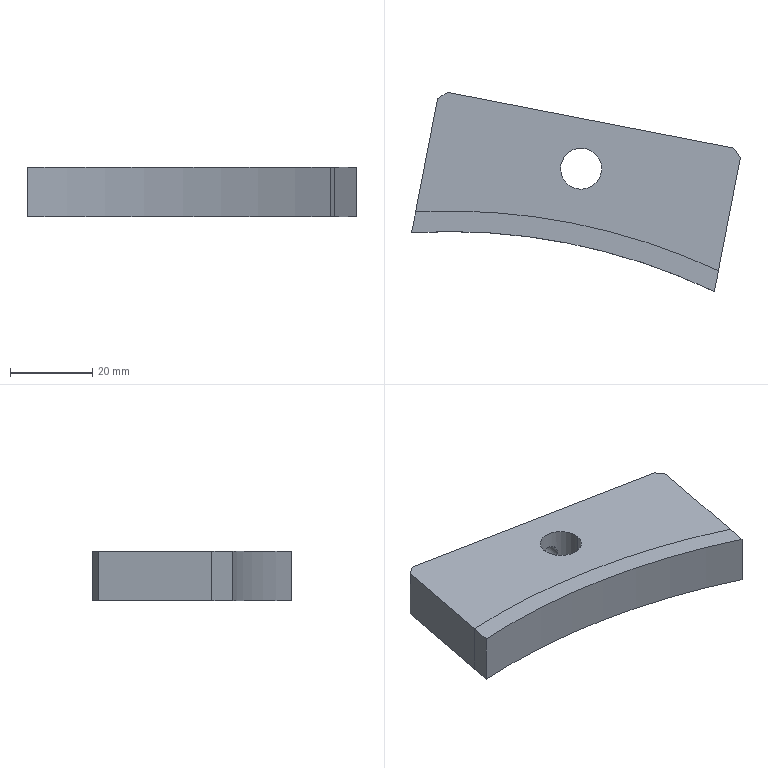Component | SolidWorks | JYTBJ-HeaderPlateBrakePad-1 | 2 solids | 18 faces | box 79.95 x 48.45 x 12 mm | volume 27686 mm3 | plane 11 | cylinder 7 | commonest cylinder face diameters 310 x2 4.2 x2 10 x2 300 x1
build123d program:
from build123d import *

# Parameters (mm, degrees)
BOSS_EXTRUDE1_DEPTH = 12
SKETCH2_R           = 5
CUT_EXTRUDE1_DEPTH  = 12
BOSS_EXTRUDE2_DEPTH = 12
CHAMFER1_SIZE       = 2


with BuildPart() as part:
    # Sketch1 → Boss-Extrude1 (new body)
    with BuildSketch(Plane.XY):
        with BuildLine():
            Line((-13.101, 22.851), (61.899, 22.851))
            Line((61.899, 22.851), (61.899, -7.149))
            ThreePointArc((61.899, -7.149), (24.399, -2.544), (-13.101, -7.149))
            Line((-13.101, -7.149), (-13.101, 22.851))
        make_face()
    extrude(amount=BOSS_EXTRUDE1_DEPTH)

    # Sketch2 → Cut-Extrude1 (cut)
    with BuildSketch(Plane.XY.offset(12)):
        with Locations((24.399, 10.851)):
            Circle(SKETCH2_R)
    extrude(amount=-CUT_EXTRUDE1_DEPTH, mode=Mode.SUBTRACT)

    # Sketch4 → M5 Tapped Hole1 (revolve, cut)
    with BuildSketch(Plane(origin=(24.399, 22.851, 6), x_dir=(0, 0, 1), z_dir=(1, 0, 0))):
        Polygon((0, 0), (0, 15.262), (2.1, 14), (2.1, 0), align=None)
    revolve(axis=Axis((24.399, 29.201, 6), (0, -1, 0)), mode=Mode.SUBTRACT)

    # Chamfer1
    chamfer1_edges = [part.edges().sort_by_distance(p)[0] for p in [
        (-13.101, 22.851, 6),
        (61.899, 22.851, 6),
    ]]
    chamfer(chamfer1_edges, length=CHAMFER1_SIZE)


with BuildPart() as body_2:
    # Sketch3 → Boss-Extrude2 (new body)
    with BuildSketch(Plane.XY.offset(12)):
        with BuildLine():
            Line((-13.101, -7.149), (-13.101, -12.307))
            ThreePointArc((-13.101, -12.307), (24.399, -7.544), (61.899, -12.307))
            Line((61.899, -12.307), (61.899, -7.149))
            ThreePointArc((61.899, -7.149), (24.399, -2.544), (-13.101, -7.149))
        make_face()
    extrude(amount=-BOSS_EXTRUDE2_DEPTH)


solid = Compound([part.part, body_2.part])

# Placed as in the assembly
solid = solid.moved(Location((9.701, 259.155, 38.5), (0, 0, -11.011)))
STEP:
#1=COLOUR_RGB('',0.7922,0.8196,0.9333);
#2=FILL_AREA_STYLE_COLOUR('',#1);
#3=FILL_AREA_STYLE('',(#2));
#4=SURFACE_STYLE_FILL_AREA(#3);
#5=SURFACE_SIDE_STYLE('',(#4));
#6=SURFACE_STYLE_USAGE(.BOTH.,#5);
#7=PRESENTATION_STYLE_ASSIGNMENT((#6));
#8=CARTESIAN_POINT('',(2.72,9.461,1.988));
#9=VERTEX_POINT('',#8);
#10=CARTESIAN_POINT('',(-0.1781,10.025,1.988));
#11=VERTEX_POINT('',#10);
#12=CARTESIAN_POINT('',(0.1402,3.931,1.988));
#13=DIRECTION('',(-0.,-0.,1.));
#14=DIRECTION('',(0.9816,-0.191,0.));
#15=AXIS2_PLACEMENT_3D('',#12,#13,#14);
#16=CIRCLE('',#15,6.102);
#17=EDGE_CURVE('',#9,#11,#16,.T.);
#18=ORIENTED_EDGE('',*,*,#17,.F.);
#19=CARTESIAN_POINT('',(2.72,9.461,1.516));
#20=VERTEX_POINT('',#19);
#21=CARTESIAN_POINT('',(2.72,9.461,1.516));
#22=DIRECTION('',(-0.,-0.,1.));
#23=VECTOR('',#22,39.37);
#24=LINE('',#21,#23);
#25=EDGE_CURVE('',#20,#9,#24,.T.);
#26=ORIENTED_EDGE('',*,*,#25,.F.);
#27=CARTESIAN_POINT('',(-0.1781,10.025,1.516));
#28=VERTEX_POINT('',#27);
#29=CARTESIAN_POINT('',(0.1402,3.931,1.516));
#30=DIRECTION('',(-0.,-0.,1.));
#31=DIRECTION('',(0.9816,-0.191,0.));
#32=AXIS2_PLACEMENT_3D('',#29,#30,#31);
#33=CIRCLE('',#32,6.102);
#34=EDGE_CURVE('',#20,#28,#33,.T.);
#35=ORIENTED_EDGE('',*,*,#34,.T.);
#36=CARTESIAN_POINT('',(-0.1781,10.025,1.516));
#37=DIRECTION('',(-0.,-0.,1.));
#38=VECTOR('',#37,39.37);
#39=LINE('',#36,#38);
#40=EDGE_CURVE('',#28,#11,#39,.T.);
#41=ORIENTED_EDGE('',*,*,#40,.T.);
#42=EDGE_LOOP('',(#18,#26,#35,#41));
#43=FACE_OUTER_BOUND('',#42,.T.);
#44=CARTESIAN_POINT('',(0.1402,3.931,1.516));
#45=DIRECTION('',(-0.,-0.,1.));
#46=DIRECTION('',(0.9816,-0.191,0.));
#47=AXIS2_PLACEMENT_3D('',#44,#45,#46);
#48=CYLINDRICAL_SURFACE('',#47,6.102);
#49=ADVANCED_FACE('',(#43),#48,.T.);
#50=CARTESIAN_POINT('',(2.682,9.262,1.988));
#51=VERTEX_POINT('',#50);
#52=CARTESIAN_POINT('',(2.72,9.461,1.988));
#53=DIRECTION('',(0.191,0.9816,0.));
#54=VECTOR('',#53,39.37);
#55=LINE('',#52,#54);
#56=EDGE_CURVE('',#51,#9,#55,.T.);
#57=ORIENTED_EDGE('',*,*,#56,.F.);
#58=CARTESIAN_POINT('',(2.682,9.262,1.516));
#59=VERTEX_POINT('',#58);
#60=CARTESIAN_POINT('',(2.682,9.262,1.516));
#61=DIRECTION('',(-0.,-0.,1.));
#62=VECTOR('',#61,39.37);
#63=LINE('',#60,#62);
#64=EDGE_CURVE('',#59,#51,#63,.T.);
#65=ORIENTED_EDGE('',*,*,#64,.F.);
#66=CARTESIAN_POINT('',(2.72,9.461,1.516));
#67=DIRECTION('',(0.191,0.9816,0.));
#68=VECTOR('',#67,39.37);
#69=LINE('',#66,#68);
#70=EDGE_CURVE('',#59,#20,#69,.T.);
#71=ORIENTED_EDGE('',*,*,#70,.T.);
#72=ORIENTED_EDGE('',*,*,#25,.T.);
#73=EDGE_LOOP('',(#57,#65,#71,#72));
#74=FACE_OUTER_BOUND('',#73,.T.);
#75=CARTESIAN_POINT('',(2.72,9.461,1.516));
#76=DIRECTION('',(0.9816,-0.191,0.));
#77=DIRECTION('',(0.,0.,-1.));
#78=AXIS2_PLACEMENT_3D('',#75,#76,#77);
#79=PLANE('',#78);
#80=ADVANCED_FACE('',(#74),#79,.T.);
#81=CARTESIAN_POINT('',(-0.2169,9.826,1.988));
#82=VERTEX_POINT('',#81);
#83=CARTESIAN_POINT('',(0.1402,3.931,1.988));
#84=DIRECTION('',(0.,0.,-1.));
#85=DIRECTION('',(0.9816,-0.191,0.));
#86=AXIS2_PLACEMENT_3D('',#83,#84,#85);
#87=CIRCLE('',#86,5.906);
#88=EDGE_CURVE('',#82,#51,#87,.T.);
#89=ORIENTED_EDGE('',*,*,#88,.F.);
#90=CARTESIAN_POINT('',(-0.2169,9.826,1.516));
#91=VERTEX_POINT('',#90);
#92=CARTESIAN_POINT('',(-0.2169,9.826,1.516));
#93=DIRECTION('',(-0.,-0.,1.));
#94=VECTOR('',#93,39.37);
#95=LINE('',#92,#94);
#96=EDGE_CURVE('',#91,#82,#95,.T.);
#97=ORIENTED_EDGE('',*,*,#96,.F.);
#98=CARTESIAN_POINT('',(0.1402,3.931,1.516));
#99=DIRECTION('',(0.,0.,-1.));
#100=DIRECTION('',(0.9816,-0.191,0.));
#101=AXIS2_PLACEMENT_3D('',#98,#99,#100);
#102=CIRCLE('',#101,5.906);
#103=EDGE_CURVE('',#91,#59,#102,.T.);
#104=ORIENTED_EDGE('',*,*,#103,.T.);
#105=ORIENTED_EDGE('',*,*,#64,.T.);
#106=EDGE_LOOP('',(#89,#97,#104,#105));
#107=FACE_OUTER_BOUND('',#106,.T.);
#108=CARTESIAN_POINT('',(0.1402,3.931,1.516));
#109=DIRECTION('',(-0.,-0.,1.));
#110=DIRECTION('',(0.9816,-0.191,0.));
#111=AXIS2_PLACEMENT_3D('',#108,#109,#110);
#112=CYLINDRICAL_SURFACE('',#111,5.906);
#113=ADVANCED_FACE('',(#107),#112,.F.);
#114=CARTESIAN_POINT('',(-0.1781,10.025,1.988));
#115=DIRECTION('',(-0.191,-0.9816,-0.));
#116=VECTOR('',#115,39.37);
#117=LINE('',#114,#116);
#118=EDGE_CURVE('',#11,#82,#117,.T.);
#119=ORIENTED_EDGE('',*,*,#118,.F.);
#120=ORIENTED_EDGE('',*,*,#40,.F.);
#121=CARTESIAN_POINT('',(-0.1781,10.025,1.516));
#122=DIRECTION('',(-0.191,-0.9816,-0.));
#123=VECTOR('',#122,39.37);
#124=LINE('',#121,#123);
#125=EDGE_CURVE('',#28,#91,#124,.T.);
#126=ORIENTED_EDGE('',*,*,#125,.T.);
#127=ORIENTED_EDGE('',*,*,#96,.T.);
#128=EDGE_LOOP('',(#119,#120,#126,#127));
#129=FACE_OUTER_BOUND('',#128,.T.);
#130=CARTESIAN_POINT('',(-0.1781,10.025,1.516));
#131=DIRECTION('',(-0.9816,0.191,-0.));
#132=DIRECTION('',(-0.191,-0.9816,-0.));
#133=AXIS2_PLACEMENT_3D('',#130,#131,#132);
#134=PLANE('',#133);
#135=ADVANCED_FACE('',(#129),#134,.T.);
#136=ORIENTED_EDGE('',*,*,#34,.F.);
#137=ORIENTED_EDGE('',*,*,#70,.F.);
#138=ORIENTED_EDGE('',*,*,#103,.F.);
#139=ORIENTED_EDGE('',*,*,#125,.F.);
#140=EDGE_LOOP('',(#136,#137,#138,#139));
#141=FACE_OUTER_BOUND('',#140,.T.);
#142=CARTESIAN_POINT('',(0.1402,3.931,1.516));
#143=DIRECTION('',(-0.,-0.,1.));
#144=DIRECTION('',(0.9816,-0.191,0.));
#145=AXIS2_PLACEMENT_3D('',#142,#143,#144);
#146=PLANE('',#145);
#147=ADVANCED_FACE('',(#141),#146,.F.);
#148=ORIENTED_EDGE('',*,*,#17,.T.);
#149=ORIENTED_EDGE('',*,*,#118,.T.);
#150=ORIENTED_EDGE('',*,*,#88,.T.);
#151=ORIENTED_EDGE('',*,*,#56,.T.);
#152=EDGE_LOOP('',(#148,#149,#150,#151));
#153=FACE_OUTER_BOUND('',#152,.T.);
#154=CARTESIAN_POINT('',(0.1402,3.931,1.988));
#155=DIRECTION('',(-0.,-0.,1.));
#156=DIRECTION('',(0.9816,-0.191,0.));
#157=AXIS2_PLACEMENT_3D('',#154,#155,#156);
#158=PLANE('',#157);
#159=ADVANCED_FACE('',(#153),#158,.T.);
#160=CLOSED_SHELL('',(#49,#80,#113,#135,#147,#159));
#161=MANIFOLD_SOLID_BREP('',#160);
#162=STYLED_ITEM('',(#7),#161);
#163=PRESENTATION_LAYER_ASSIGNMENT('','',(#162));
#164=COLOUR_RGB('',0.7922,0.8196,0.9333);
#165=FILL_AREA_STYLE_COLOUR('',#164);
#166=FILL_AREA_STYLE('',(#165));
#167=SURFACE_STYLE_FILL_AREA(#166);
#168=SURFACE_SIDE_STYLE('',(#167));
#169=SURFACE_STYLE_USAGE(.BOTH.,#168);
#170=PRESENTATION_STYLE_ASSIGNMENT((#169));
#171=CARTESIAN_POINT('',(1.444,10.632,1.669));
#172=VERTEX_POINT('',#171);
#173=CARTESIAN_POINT('',(1.444,10.632,1.835));
#174=VERTEX_POINT('',#173);
#175=CARTESIAN_POINT('',(1.444,10.632,1.669));
#176=CARTESIAN_POINT('',(1.439,10.633,1.669));
#177=CARTESIAN_POINT('',(1.433,10.634,1.67));
#178=CARTESIAN_POINT('',(1.423,10.635,1.672));
#179=CARTESIAN_POINT('',(1.417,10.635,1.674));
#180=CARTESIAN_POINT('',(1.407,10.636,1.678));
#181=CARTESIAN_POINT('',(1.402,10.636,1.68));
#182=CARTESIAN_POINT('',(1.393,10.635,1.686));
#183=CARTESIAN_POINT('',(1.389,10.635,1.69));
#184=CARTESIAN_POINT('',(1.381,10.634,1.697));
#185=CARTESIAN_POINT('',(1.377,10.634,1.701));
#186=CARTESIAN_POINT('',(1.371,10.633,1.71));
#187=CARTESIAN_POINT('',(1.368,10.632,1.715));
#188=CARTESIAN_POINT('',(1.364,10.631,1.725));
#189=CARTESIAN_POINT('',(1.362,10.631,1.73));
#190=CARTESIAN_POINT('',(1.36,10.63,1.741));
#191=CARTESIAN_POINT('',(1.359,10.63,1.746));
#192=CARTESIAN_POINT('',(1.359,10.63,1.763));
#193=CARTESIAN_POINT('',(1.362,10.631,1.774));
#194=CARTESIAN_POINT('',(1.368,10.632,1.789));
#195=CARTESIAN_POINT('',(1.371,10.633,1.794));
#196=CARTESIAN_POINT('',(1.377,10.634,1.802));
#197=CARTESIAN_POINT('',(1.381,10.634,1.807));
#198=CARTESIAN_POINT('',(1.389,10.635,1.814));
#199=CARTESIAN_POINT('',(1.393,10.635,1.818));
#200=CARTESIAN_POINT('',(1.402,10.636,1.824));
#201=CARTESIAN_POINT('',(1.407,10.636,1.826));
#202=CARTESIAN_POINT('',(1.417,10.635,1.83));
#203=CARTESIAN_POINT('',(1.423,10.635,1.832));
#204=CARTESIAN_POINT('',(1.433,10.634,1.834));
#205=CARTESIAN_POINT('',(1.439,10.633,1.835));
#206=CARTESIAN_POINT('',(1.444,10.632,1.835));
#207=B_SPLINE_CURVE_WITH_KNOTS('',3,(#175,#176,#177,#178,#179,#180,#181,#182,#183,#184,#185,#186,#187,#188,#189,#190,#191,#192,#193,#194,#195,#196,#197,#198,#199,#200,#201,#202,#203,#204,#205,#206),.UNSPECIFIED.,.F.,.F.,(4,2,2,2,2,2,2,2,2,2,2,2,2,2,2,4),(0.006644,0.007058,0.007473,0.007888,0.008303,0.008718,0.009133,0.009548,0.009963,0.01079,0.01121,0.01162,0.01204,0.01245,0.01287,0.01328),.UNSPECIFIED.);
#208=EDGE_CURVE('',#172,#174,#207,.T.);
#209=ORIENTED_EDGE('',*,*,#208,.F.);
#210=CARTESIAN_POINT('',(1.497,10.903,1.669));
#211=VERTEX_POINT('',#210);
#212=CARTESIAN_POINT('',(1.497,10.903,1.669));
#213=DIRECTION('',(0.191,0.9816,0.));
#214=VECTOR('',#213,39.37);
#215=LINE('',#212,#214);
#216=EDGE_CURVE('',#172,#211,#215,.T.);
#217=ORIENTED_EDGE('',*,*,#216,.T.);
#218=CARTESIAN_POINT('',(1.497,10.903,1.835));
#219=VERTEX_POINT('',#218);
#220=CARTESIAN_POINT('',(1.497,10.903,1.752));
#221=DIRECTION('',(0.191,0.9816,0.));
#222=DIRECTION('',(0.,0.,1.));
#223=AXIS2_PLACEMENT_3D('',#220,#221,#222);
#224=CIRCLE('',#223,0.08268);
#225=EDGE_CURVE('',#211,#219,#224,.T.);
#226=ORIENTED_EDGE('',*,*,#225,.T.);
#227=CARTESIAN_POINT('',(1.497,10.903,1.835));
#228=DIRECTION('',(0.191,0.9816,0.));
#229=VECTOR('',#228,39.37);
#230=LINE('',#227,#229);
#231=EDGE_CURVE('',#174,#219,#230,.T.);
#232=ORIENTED_EDGE('',*,*,#231,.F.);
#233=EDGE_LOOP('',(#209,#217,#226,#232));
#234=FACE_OUTER_BOUND('',#233,.T.);
#235=CARTESIAN_POINT('',(1.497,10.903,1.752));
#236=DIRECTION('',(0.191,0.9816,0.));
#237=DIRECTION('',(0.,0.,1.));
#238=AXIS2_PLACEMENT_3D('',#235,#236,#237);
#239=CYLINDRICAL_SURFACE('',#238,0.08268);
#240=ADVANCED_FACE('',(#234),#239,.F.);
#241=CARTESIAN_POINT('',(1.213,10.476,1.516));
#242=VERTEX_POINT('',#241);
#243=CARTESIAN_POINT('',(1.6,10.401,1.516));
#244=VERTEX_POINT('',#243);
#245=CARTESIAN_POINT('',(1.406,10.439,1.516));
#246=DIRECTION('',(-0.,-0.,1.));
#247=DIRECTION('',(0.9816,-0.191,0.));
#248=AXIS2_PLACEMENT_3D('',#245,#246,#247);
#249=CIRCLE('',#248,0.1969);
#250=EDGE_CURVE('',#242,#244,#249,.T.);
#251=ORIENTED_EDGE('',*,*,#250,.F.);
#252=CARTESIAN_POINT('',(1.213,10.476,1.988));
#253=VERTEX_POINT('',#252);
#254=CARTESIAN_POINT('',(1.213,10.476,1.516));
#255=DIRECTION('',(-0.,-0.,1.));
#256=VECTOR('',#255,39.37);
#257=LINE('',#254,#256);
#258=EDGE_CURVE('',#242,#253,#257,.T.);
#259=ORIENTED_EDGE('',*,*,#258,.T.);
#260=CARTESIAN_POINT('',(1.6,10.401,1.988));
#261=VERTEX_POINT('',#260);
#262=CARTESIAN_POINT('',(1.406,10.439,1.988));
#263=DIRECTION('',(-0.,-0.,1.));
#264=DIRECTION('',(0.9816,-0.191,0.));
#265=AXIS2_PLACEMENT_3D('',#262,#263,#264);
#266=CIRCLE('',#265,0.1969);
#267=EDGE_CURVE('',#253,#261,#266,.T.);
#268=ORIENTED_EDGE('',*,*,#267,.T.);
#269=CARTESIAN_POINT('',(1.6,10.401,1.516));
#270=DIRECTION('',(-0.,-0.,1.));
#271=VECTOR('',#270,39.37);
#272=LINE('',#269,#271);
#273=EDGE_CURVE('',#244,#261,#272,.T.);
#274=ORIENTED_EDGE('',*,*,#273,.F.);
#275=EDGE_LOOP('',(#251,#259,#268,#274));
#276=FACE_OUTER_BOUND('',#275,.T.);
#277=CARTESIAN_POINT('',(1.406,10.439,1.516));
#278=DIRECTION('',(-0.,-0.,1.));
#279=DIRECTION('',(0.9816,-0.191,0.));
#280=AXIS2_PLACEMENT_3D('',#277,#278,#279);
#281=CYLINDRICAL_SURFACE('',#280,0.1969);
#282=ADVANCED_FACE('',(#276),#281,.F.);
#283=CARTESIAN_POINT('',(0.03244,11.107,1.988));
#284=VERTEX_POINT('',#283);
#285=CARTESIAN_POINT('',(-0.1781,10.025,1.988));
#286=VERTEX_POINT('',#285);
#287=CARTESIAN_POINT('',(0.04748,11.185,1.988));
#288=DIRECTION('',(-0.191,-0.9816,-0.));
#289=VECTOR('',#288,39.37);
#290=LINE('',#287,#289);
#291=EDGE_CURVE('',#284,#286,#290,.T.);
#292=ORIENTED_EDGE('',*,*,#291,.F.);
#293=CARTESIAN_POINT('',(0.03244,11.107,1.516));
#294=VERTEX_POINT('',#293);
#295=CARTESIAN_POINT('',(0.03244,11.107,1.988));
#296=DIRECTION('',(0.,0.,-1.));
#297=VECTOR('',#296,39.37);
#298=LINE('',#295,#297);
#299=EDGE_CURVE('',#284,#294,#298,.T.);
#300=ORIENTED_EDGE('',*,*,#299,.T.);
#301=CARTESIAN_POINT('',(-0.1781,10.025,1.516));
#302=VERTEX_POINT('',#301);
#303=CARTESIAN_POINT('',(0.04748,11.185,1.516));
#304=DIRECTION('',(-0.191,-0.9816,-0.));
#305=VECTOR('',#304,39.37);
#306=LINE('',#303,#305);
#307=EDGE_CURVE('',#294,#302,#306,.T.);
#308=ORIENTED_EDGE('',*,*,#307,.T.);
#309=CARTESIAN_POINT('',(-0.1781,10.025,1.988));
#310=DIRECTION('',(0.,0.,-1.));
#311=VECTOR('',#310,39.37);
#312=LINE('',#309,#311);
#313=EDGE_CURVE('',#286,#302,#312,.T.);
#314=ORIENTED_EDGE('',*,*,#313,.F.);
#315=EDGE_LOOP('',(#292,#300,#308,#314));
#316=FACE_OUTER_BOUND('',#315,.T.);
#317=CARTESIAN_POINT('',(0.04748,11.185,1.988));
#318=DIRECTION('',(0.9816,-0.191,0.));
#319=DIRECTION('',(0.191,0.9816,0.));
#320=AXIS2_PLACEMENT_3D('',#317,#318,#319);
#321=PLANE('',#320);
#322=ADVANCED_FACE('',(#316),#321,.F.);
#323=CARTESIAN_POINT('',(2.72,9.461,1.516));
#324=VERTEX_POINT('',#323);
#325=CARTESIAN_POINT('',(0.1402,3.931,1.516));
#326=DIRECTION('',(0.,0.,-1.));
#327=DIRECTION('',(0.9816,-0.191,0.));
#328=AXIS2_PLACEMENT_3D('',#325,#326,#327);
#329=CIRCLE('',#328,6.102);
#330=EDGE_CURVE('',#302,#324,#329,.T.);
#331=ORIENTED_EDGE('',*,*,#330,.T.);
#332=CARTESIAN_POINT('',(2.72,9.461,1.988));
#333=VERTEX_POINT('',#332);
#334=CARTESIAN_POINT('',(2.72,9.461,1.988));
#335=DIRECTION('',(0.,0.,-1.));
#336=VECTOR('',#335,39.37);
#337=LINE('',#334,#336);
#338=EDGE_CURVE('',#333,#324,#337,.T.);
#339=ORIENTED_EDGE('',*,*,#338,.F.);
#340=CARTESIAN_POINT('',(0.1402,3.931,1.988));
#341=DIRECTION('',(0.,0.,-1.));
#342=DIRECTION('',(0.9816,-0.191,0.));
#343=AXIS2_PLACEMENT_3D('',#340,#341,#342);
#344=CIRCLE('',#343,6.102);
#345=EDGE_CURVE('',#286,#333,#344,.T.);
#346=ORIENTED_EDGE('',*,*,#345,.F.);
#347=ORIENTED_EDGE('',*,*,#313,.T.);
#348=EDGE_LOOP('',(#331,#339,#346,#347));
#349=FACE_OUTER_BOUND('',#348,.T.);
#350=CARTESIAN_POINT('',(0.1402,3.931,1.988));
#351=DIRECTION('',(0.,0.,-1.));
#352=DIRECTION('',(-0.9816,0.191,0.));
#353=AXIS2_PLACEMENT_3D('',#350,#351,#352);
#354=CYLINDRICAL_SURFACE('',#353,6.102);
#355=ADVANCED_FACE('',(#349),#354,.F.);
#356=CARTESIAN_POINT('',(2.931,10.543,1.516));
#357=VERTEX_POINT('',#356);
#358=CARTESIAN_POINT('',(2.946,10.621,1.516));
#359=DIRECTION('',(0.191,0.9816,0.));
#360=VECTOR('',#359,39.37);
#361=LINE('',#358,#360);
#362=EDGE_CURVE('',#324,#357,#361,.T.);
#363=ORIENTED_EDGE('',*,*,#362,.T.);
#364=CARTESIAN_POINT('',(2.931,10.543,1.988));
#365=VERTEX_POINT('',#364);
#366=CARTESIAN_POINT('',(2.931,10.543,1.988));
#367=DIRECTION('',(-0.,-0.,1.));
#368=VECTOR('',#367,39.37);
#369=LINE('',#366,#368);
#370=EDGE_CURVE('',#357,#365,#369,.T.);
#371=ORIENTED_EDGE('',*,*,#370,.T.);
#372=CARTESIAN_POINT('',(2.946,10.621,1.988));
#373=DIRECTION('',(0.191,0.9816,0.));
#374=VECTOR('',#373,39.37);
#375=LINE('',#372,#374);
#376=EDGE_CURVE('',#333,#365,#375,.T.);
#377=ORIENTED_EDGE('',*,*,#376,.F.);
#378=ORIENTED_EDGE('',*,*,#338,.T.);
#379=EDGE_LOOP('',(#363,#371,#377,#378));
#380=FACE_OUTER_BOUND('',#379,.T.);
#381=CARTESIAN_POINT('',(2.946,10.621,1.988));
#382=DIRECTION('',(-0.9816,0.191,-0.));
#383=DIRECTION('',(-0.,-0.,1.));
#384=AXIS2_PLACEMENT_3D('',#381,#382,#383);
#385=PLANE('',#384);
#386=ADVANCED_FACE('',(#380),#385,.F.);
#387=CARTESIAN_POINT('',(1.497,10.903,1.752));
#388=DIRECTION('',(0.191,0.9816,0.));
#389=DIRECTION('',(0.,0.,1.));
#390=AXIS2_PLACEMENT_3D('',#387,#388,#389);
#391=CIRCLE('',#390,0.08268);
#392=EDGE_CURVE('',#219,#211,#391,.T.);
#393=ORIENTED_EDGE('',*,*,#392,.F.);
#394=ORIENTED_EDGE('',*,*,#225,.F.);
#395=EDGE_LOOP('',(#393,#394));
#396=FACE_BOUND('',#395,.T.);
#397=CARTESIAN_POINT('',(2.869,10.636,1.988));
#398=VERTEX_POINT('',#397);
#399=CARTESIAN_POINT('',(0.1248,11.17,1.988));
#400=VERTEX_POINT('',#399);
#401=CARTESIAN_POINT('',(0.04748,11.185,1.988));
#402=DIRECTION('',(-0.9816,0.191,-0.));
#403=VECTOR('',#402,39.37);
#404=LINE('',#401,#403);
#405=EDGE_CURVE('',#398,#400,#404,.T.);
#406=ORIENTED_EDGE('',*,*,#405,.F.);
#407=CARTESIAN_POINT('',(2.869,10.636,1.516));
#408=VERTEX_POINT('',#407);
#409=CARTESIAN_POINT('',(2.869,10.636,1.988));
#410=DIRECTION('',(0.,0.,-1.));
#411=VECTOR('',#410,39.37);
#412=LINE('',#409,#411);
#413=EDGE_CURVE('',#398,#408,#412,.T.);
#414=ORIENTED_EDGE('',*,*,#413,.T.);
#415=CARTESIAN_POINT('',(0.1248,11.17,1.516));
#416=VERTEX_POINT('',#415);
#417=CARTESIAN_POINT('',(0.04748,11.185,1.516));
#418=DIRECTION('',(-0.9816,0.191,-0.));
#419=VECTOR('',#418,39.37);
#420=LINE('',#417,#419);
#421=EDGE_CURVE('',#408,#416,#420,.T.);
#422=ORIENTED_EDGE('',*,*,#421,.T.);
#423=CARTESIAN_POINT('',(0.1248,11.17,1.988));
#424=DIRECTION('',(-0.,-0.,1.));
#425=VECTOR('',#424,39.37);
#426=LINE('',#423,#425);
#427=EDGE_CURVE('',#416,#400,#426,.T.);
#428=ORIENTED_EDGE('',*,*,#427,.T.);
#429=EDGE_LOOP('',(#406,#414,#422,#428));
#430=FACE_OUTER_BOUND('',#429,.T.);
#431=CARTESIAN_POINT('',(0.04748,11.185,1.988));
#432=DIRECTION('',(-0.191,-0.9816,-0.));
#433=DIRECTION('',(0.,0.,-1.));
#434=AXIS2_PLACEMENT_3D('',#431,#432,#433);
#435=PLANE('',#434);
#436=ADVANCED_FACE('',(#396,#430),#435,.F.);
#437=CARTESIAN_POINT('',(1.406,10.439,1.988));
#438=DIRECTION('',(-0.,-0.,1.));
#439=DIRECTION('',(0.9816,-0.191,0.));
#440=AXIS2_PLACEMENT_3D('',#437,#438,#439);
#441=CIRCLE('',#440,0.1969);
#442=EDGE_CURVE('',#261,#253,#441,.T.);
#443=ORIENTED_EDGE('',*,*,#442,.F.);
#444=ORIENTED_EDGE('',*,*,#267,.F.);
#445=EDGE_LOOP('',(#443,#444));
#446=FACE_BOUND('',#445,.T.);
#447=ORIENTED_EDGE('',*,*,#376,.T.);
#448=CARTESIAN_POINT('',(5.124,7.291,1.988));
#449=DIRECTION('',(-0.559,0.8291,0.));
#450=VECTOR('',#449,39.37);
#451=LINE('',#448,#450);
#452=EDGE_CURVE('',#365,#398,#451,.T.);
#453=ORIENTED_EDGE('',*,*,#452,.T.);
#454=ORIENTED_EDGE('',*,*,#405,.T.);
#455=CARTESIAN_POINT('',(-3.22,8.915,1.988));
#456=DIRECTION('',(-0.8291,-0.559,-0.));
#457=VECTOR('',#456,39.37);
#458=LINE('',#455,#457);
#459=EDGE_CURVE('',#400,#284,#458,.T.);
#460=ORIENTED_EDGE('',*,*,#459,.T.);
#461=ORIENTED_EDGE('',*,*,#291,.T.);
#462=ORIENTED_EDGE('',*,*,#345,.T.);
#463=EDGE_LOOP('',(#447,#453,#454,#460,#461,#462));
#464=FACE_OUTER_BOUND('',#463,.T.);
#465=CARTESIAN_POINT('',(0.1402,3.931,1.988));
#466=DIRECTION('',(-0.,-0.,1.));
#467=DIRECTION('',(0.9816,-0.191,0.));
#468=AXIS2_PLACEMENT_3D('',#465,#466,#467);
#469=PLANE('',#468);
#470=ADVANCED_FACE('',(#446,#464),#469,.T.);
#471=CARTESIAN_POINT('',(1.406,10.439,1.516));
#472=DIRECTION('',(-0.,-0.,1.));
#473=DIRECTION('',(0.9816,-0.191,0.));
#474=AXIS2_PLACEMENT_3D('',#471,#472,#473);
#475=CIRCLE('',#474,0.1969);
#476=EDGE_CURVE('',#244,#242,#475,.T.);
#477=ORIENTED_EDGE('',*,*,#476,.T.);
#478=ORIENTED_EDGE('',*,*,#250,.T.);
#479=EDGE_LOOP('',(#477,#478));
#480=FACE_BOUND('',#479,.T.);
#481=ORIENTED_EDGE('',*,*,#421,.F.);
#482=CARTESIAN_POINT('',(2.869,10.636,1.516));
#483=DIRECTION('',(0.559,-0.8291,-0.));
#484=VECTOR('',#483,39.37);
#485=LINE('',#482,#484);
#486=EDGE_CURVE('',#408,#357,#485,.T.);
#487=ORIENTED_EDGE('',*,*,#486,.T.);
#488=ORIENTED_EDGE('',*,*,#362,.F.);
#489=ORIENTED_EDGE('',*,*,#330,.F.);
#490=ORIENTED_EDGE('',*,*,#307,.F.);
#491=CARTESIAN_POINT('',(0.03244,11.107,1.516));
#492=DIRECTION('',(0.8291,0.559,0.));
#493=VECTOR('',#492,39.37);
#494=LINE('',#491,#493);
#495=EDGE_CURVE('',#294,#416,#494,.T.);
#496=ORIENTED_EDGE('',*,*,#495,.T.);
#497=EDGE_LOOP('',(#481,#487,#488,#489,#490,#496));
#498=FACE_OUTER_BOUND('',#497,.T.);
#499=CARTESIAN_POINT('',(0.1402,3.931,1.516));
#500=DIRECTION('',(-0.,-0.,1.));
#501=DIRECTION('',(0.9816,-0.191,0.));
#502=AXIS2_PLACEMENT_3D('',#499,#500,#501);
#503=PLANE('',#502);
#504=ADVANCED_FACE('',(#480,#498),#503,.F.);
#505=ORIENTED_EDGE('',*,*,#258,.F.);
#506=ORIENTED_EDGE('',*,*,#476,.F.);
#507=ORIENTED_EDGE('',*,*,#273,.T.);
#508=ORIENTED_EDGE('',*,*,#442,.T.);
#509=EDGE_LOOP('',(#505,#506,#507,#508));
#510=FACE_OUTER_BOUND('',#509,.T.);
#511=CARTESIAN_POINT('',(1.444,10.632,1.835));
#512=CARTESIAN_POINT('',(1.449,10.631,1.835));
#513=CARTESIAN_POINT('',(1.455,10.63,1.834));
#514=CARTESIAN_POINT('',(1.465,10.627,1.832));
#515=CARTESIAN_POINT('',(1.47,10.625,1.83));
#516=CARTESIAN_POINT('',(1.48,10.622,1.826));
#517=CARTESIAN_POINT('',(1.484,10.62,1.824));
#518=CARTESIAN_POINT('',(1.492,10.616,1.818));
#519=CARTESIAN_POINT('',(1.496,10.614,1.814));
#520=CARTESIAN_POINT('',(1.507,10.608,1.803));
#521=CARTESIAN_POINT('',(1.512,10.605,1.794));
#522=CARTESIAN_POINT('',(1.518,10.601,1.779));
#523=CARTESIAN_POINT('',(1.519,10.6,1.774));
#524=CARTESIAN_POINT('',(1.521,10.599,1.763));
#525=CARTESIAN_POINT('',(1.522,10.598,1.757));
#526=CARTESIAN_POINT('',(1.522,10.598,1.747));
#527=CARTESIAN_POINT('',(1.521,10.599,1.741));
#528=CARTESIAN_POINT('',(1.519,10.6,1.73));
#529=CARTESIAN_POINT('',(1.518,10.601,1.725));
#530=CARTESIAN_POINT('',(1.514,10.604,1.715));
#531=CARTESIAN_POINT('',(1.512,10.605,1.71));
#532=CARTESIAN_POINT('',(1.506,10.608,1.701));
#533=CARTESIAN_POINT('',(1.503,10.61,1.697));
#534=CARTESIAN_POINT('',(1.496,10.614,1.69));
#535=CARTESIAN_POINT('',(1.492,10.616,1.686));
#536=CARTESIAN_POINT('',(1.484,10.62,1.68));
#537=CARTESIAN_POINT('',(1.48,10.622,1.678));
#538=CARTESIAN_POINT('',(1.465,10.627,1.672));
#539=CARTESIAN_POINT('',(1.455,10.63,1.669));
#540=CARTESIAN_POINT('',(1.444,10.632,1.669));
#541=B_SPLINE_CURVE_WITH_KNOTS('',3,(#511,#512,#513,#514,#515,#516,#517,#518,#519,#520,#521,#522,#523,#524,#525,#526,#527,#528,#529,#530,#531,#532,#533,#534,#535,#536,#537,#538,#539,#540),.UNSPECIFIED.,.F.,.F.,(4,2,2,2,2,2,2,2,2,2,2,2,2,2,4),(0.,0.0004152,0.0008304,0.001246,0.001661,0.002491,0.002907,0.003322,0.003737,0.004152,0.004567,0.004983,0.005398,0.005813,0.006644),.UNSPECIFIED.);
#542=EDGE_CURVE('',#174,#172,#541,.T.);
#543=ORIENTED_EDGE('',*,*,#542,.T.);
#544=ORIENTED_EDGE('',*,*,#208,.T.);
#545=EDGE_LOOP('',(#543,#544));
#546=FACE_BOUND('',#545,.T.);
#547=CARTESIAN_POINT('',(1.406,10.439,1.516));
#548=DIRECTION('',(-0.,-0.,1.));
#549=DIRECTION('',(0.9816,-0.191,0.));
#550=AXIS2_PLACEMENT_3D('',#547,#548,#549);
#551=CYLINDRICAL_SURFACE('',#550,0.1969);
#552=ADVANCED_FACE('',(#510,#546),#551,.F.);
#553=ORIENTED_EDGE('',*,*,#216,.F.);
#554=ORIENTED_EDGE('',*,*,#542,.F.);
#555=ORIENTED_EDGE('',*,*,#231,.T.);
#556=ORIENTED_EDGE('',*,*,#392,.T.);
#557=EDGE_LOOP('',(#553,#554,#555,#556));
#558=FACE_OUTER_BOUND('',#557,.T.);
#559=CARTESIAN_POINT('',(1.497,10.903,1.752));
#560=DIRECTION('',(0.191,0.9816,0.));
#561=DIRECTION('',(0.,0.,1.));
#562=AXIS2_PLACEMENT_3D('',#559,#560,#561);
#563=CYLINDRICAL_SURFACE('',#562,0.08268);
#564=ADVANCED_FACE('',(#558),#563,.F.);
#565=ORIENTED_EDGE('',*,*,#452,.F.);
#566=ORIENTED_EDGE('',*,*,#370,.F.);
#567=ORIENTED_EDGE('',*,*,#486,.F.);
#568=ORIENTED_EDGE('',*,*,#413,.F.);
#569=EDGE_LOOP('',(#565,#566,#567,#568));
#570=FACE_OUTER_BOUND('',#569,.T.);
#571=CARTESIAN_POINT('',(2.869,10.636,1.988));
#572=DIRECTION('',(-0.8291,-0.559,-0.));
#573=DIRECTION('',(0.559,-0.8291,-0.));
#574=AXIS2_PLACEMENT_3D('',#571,#572,#573);
#575=PLANE('',#574);
#576=ADVANCED_FACE('',(#570),#575,.F.);
#577=ORIENTED_EDGE('',*,*,#459,.F.);
#578=ORIENTED_EDGE('',*,*,#427,.F.);
#579=ORIENTED_EDGE('',*,*,#495,.F.);
#580=ORIENTED_EDGE('',*,*,#299,.F.);
#581=EDGE_LOOP('',(#577,#578,#579,#580));
#582=FACE_OUTER_BOUND('',#581,.T.);
#583=CARTESIAN_POINT('',(0.03244,11.107,1.988));
#584=DIRECTION('',(0.559,-0.8291,-0.));
#585=DIRECTION('',(0.8291,0.559,0.));
#586=AXIS2_PLACEMENT_3D('',#583,#584,#585);
#587=PLANE('',#586);
#588=ADVANCED_FACE('',(#582),#587,.F.);
#589=CLOSED_SHELL('',(#240,#282,#322,#355,#386,#436,#470,#504,#552,#564,#576,#588));
#590=MANIFOLD_SOLID_BREP('',#589);
#591=STYLED_ITEM('',(#170),#590);
#592=(LENGTH_UNIT()NAMED_UNIT(*)SI_UNIT($,.METRE.));
#593=LENGTH_MEASURE_WITH_UNIT(LENGTH_MEASURE(0.0254),#592);
#594=DIMENSIONAL_EXPONENTS(1.,0.,0.,0.,0.,0.,0.);
#595=(CONVERSION_BASED_UNIT('',#593)LENGTH_UNIT()NAMED_UNIT(#594));
#596=UNCERTAINTY_MEASURE_WITH_UNIT(LENGTH_MEASURE(0.00001),#595,'','');
#597=(NAMED_UNIT(*)PLANE_ANGLE_UNIT()SI_UNIT($,.RADIAN.));
#598=(NAMED_UNIT(*)SI_UNIT($,.STERADIAN.)SOLID_ANGLE_UNIT());
#599=(GEOMETRIC_REPRESENTATION_CONTEXT(3)GLOBAL_UNCERTAINTY_ASSIGNED_CONTEXT((#596))GLOBAL_UNIT_ASSIGNED_CONTEXT((#595,#597,#598))REPRESENTATION_CONTEXT('',''));
#600=MECHANICAL_DESIGN_GEOMETRIC_PRESENTATION_REPRESENTATION('',(#591),#599);
#601=PRESENTATION_LAYER_ASSIGNMENT('','',(#591));
#602=CARTESIAN_POINT('',(0.,0.,0.));
#603=DIRECTION('',(0.,0.,1.));
#604=DIRECTION('',(1.,0.,0.));
#605=AXIS2_PLACEMENT_3D('',#602,#603,#604);
#606=(LENGTH_UNIT()NAMED_UNIT(*)SI_UNIT($,.METRE.));
#607=LENGTH_MEASURE_WITH_UNIT(LENGTH_MEASURE(0.0254),#606);
#608=DIMENSIONAL_EXPONENTS(1.,0.,0.,0.,0.,0.,0.);
#609=(CONVERSION_BASED_UNIT('',#607)LENGTH_UNIT()NAMED_UNIT(#608));
#610=UNCERTAINTY_MEASURE_WITH_UNIT(LENGTH_MEASURE(0.00001),#609,'','');
#611=(NAMED_UNIT(*)PLANE_ANGLE_UNIT()SI_UNIT($,.RADIAN.));
#612=(NAMED_UNIT(*)SI_UNIT($,.STERADIAN.)SOLID_ANGLE_UNIT());
#613=(GEOMETRIC_REPRESENTATION_CONTEXT(3)GLOBAL_UNCERTAINTY_ASSIGNED_CONTEXT((#610))GLOBAL_UNIT_ASSIGNED_CONTEXT((#609,#611,#612))REPRESENTATION_CONTEXT('',''));
#614=ADVANCED_BREP_SHAPE_REPRESENTATION('',(#161,#590,#605),#613);
#615=(LENGTH_UNIT()NAMED_UNIT(*)SI_UNIT($,.METRE.));
#616=LENGTH_MEASURE_WITH_UNIT(LENGTH_MEASURE(0.0254),#615);
#617=DIMENSIONAL_EXPONENTS(1.,0.,0.,0.,0.,0.,0.);
#618=(CONVERSION_BASED_UNIT('',#616)LENGTH_UNIT()NAMED_UNIT(#617));
#619=UNCERTAINTY_MEASURE_WITH_UNIT(LENGTH_MEASURE(0.00001),#618,'','');
#620=(NAMED_UNIT(*)PLANE_ANGLE_UNIT()SI_UNIT($,.RADIAN.));
#621=(NAMED_UNIT(*)SI_UNIT($,.STERADIAN.)SOLID_ANGLE_UNIT());
#622=(GEOMETRIC_REPRESENTATION_CONTEXT(3)GLOBAL_UNCERTAINTY_ASSIGNED_CONTEXT((#619))GLOBAL_UNIT_ASSIGNED_CONTEXT((#618,#620,#621))REPRESENTATION_CONTEXT('',''));
#623=MECHANICAL_DESIGN_GEOMETRIC_PRESENTATION_REPRESENTATION('',(#162),#622);